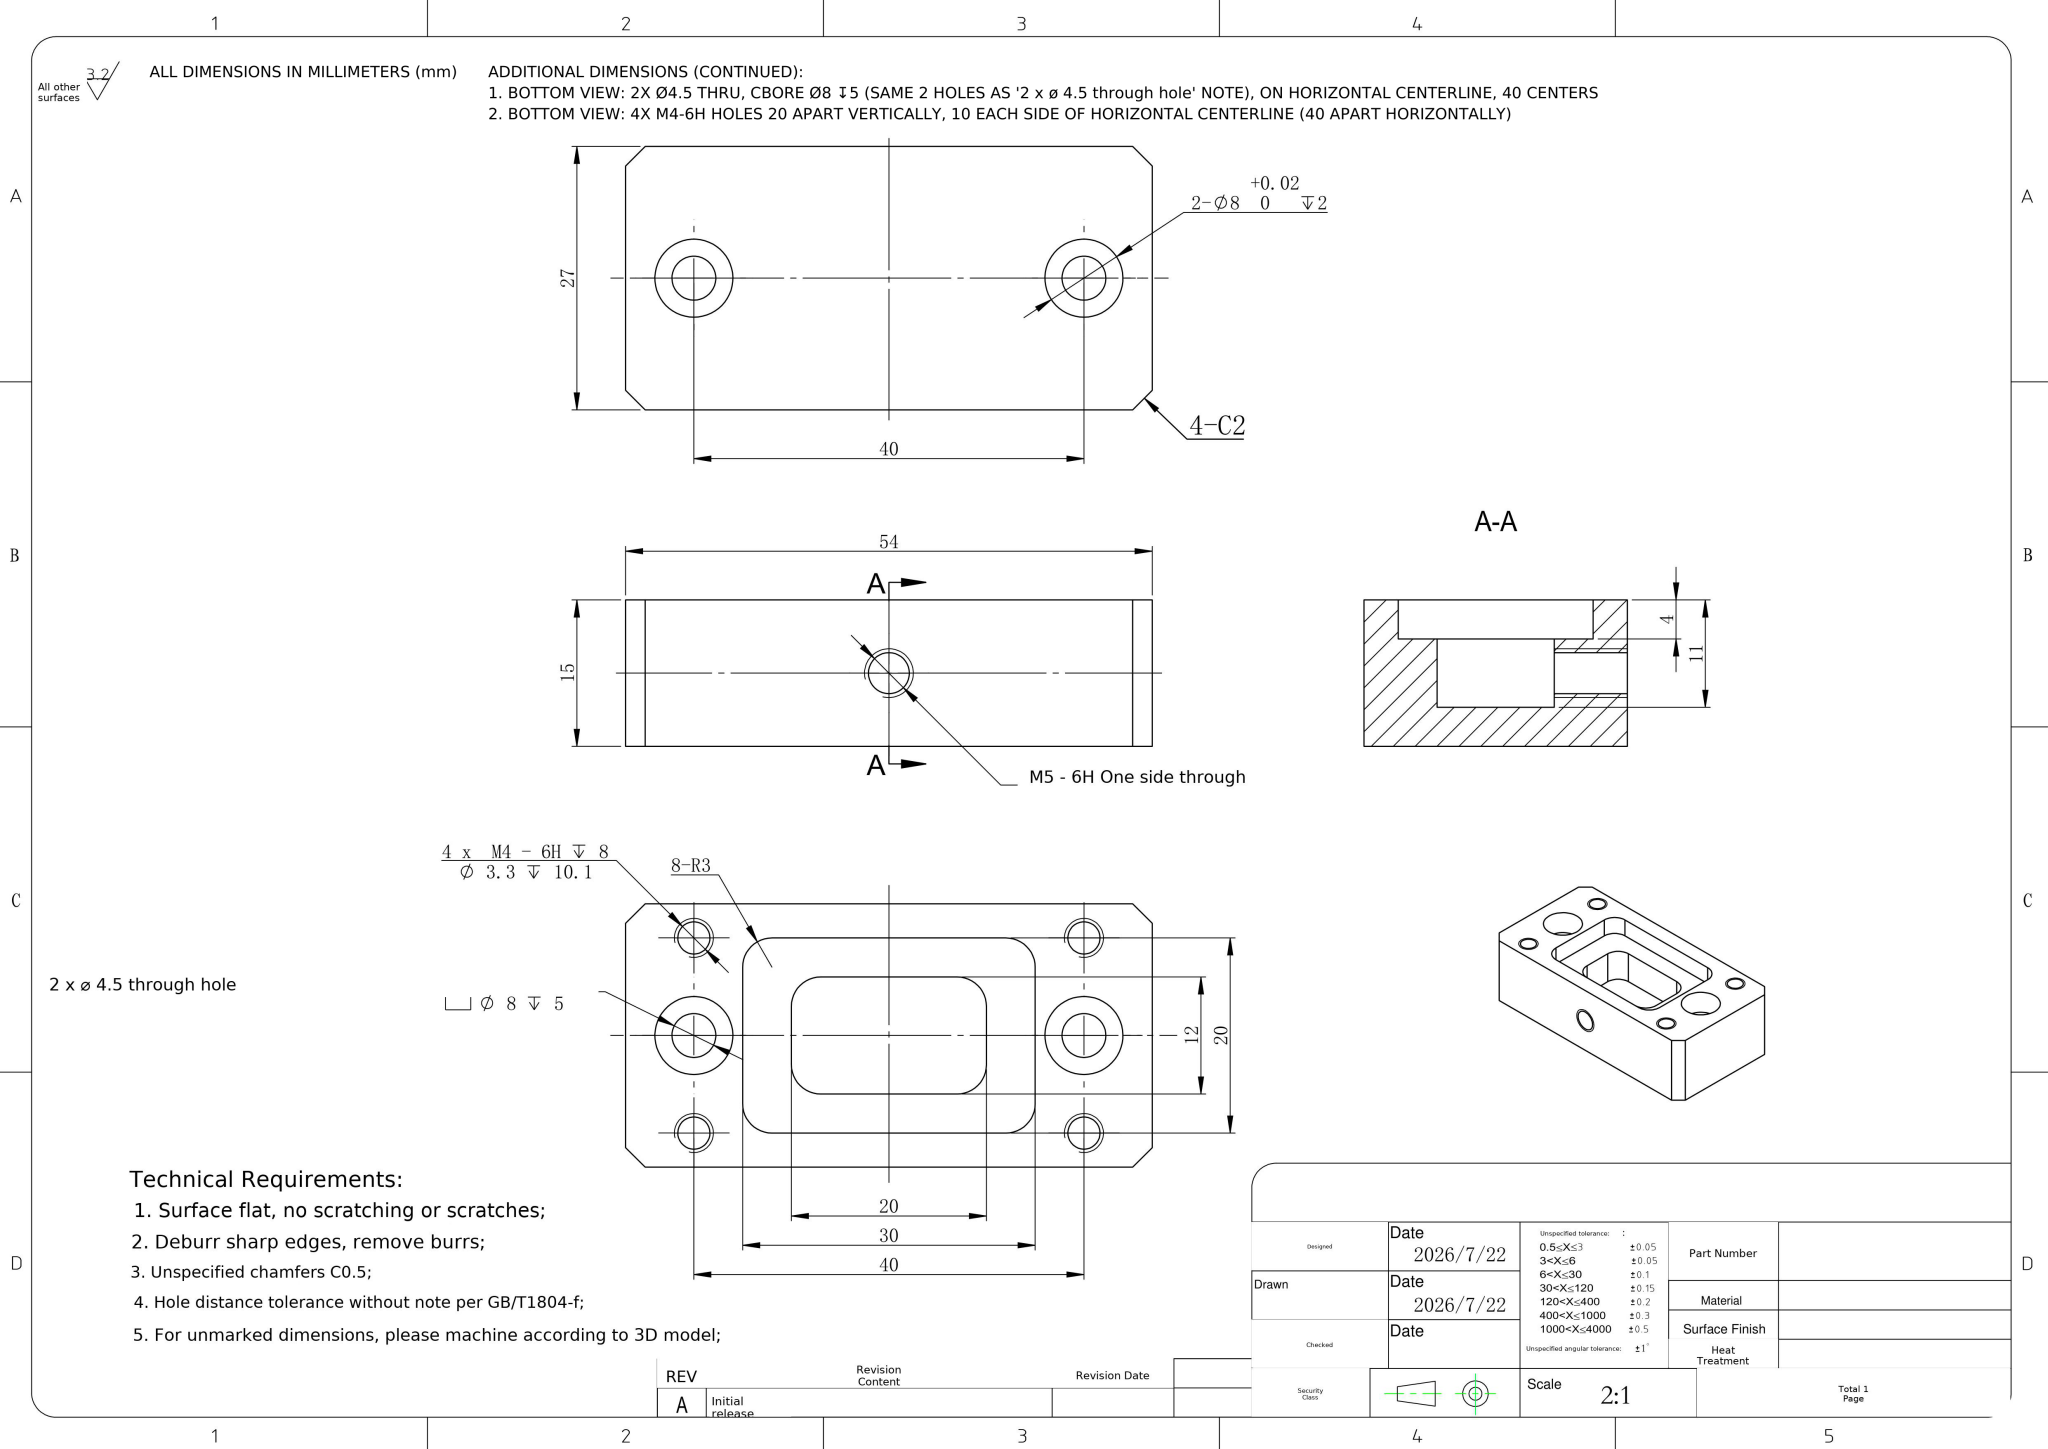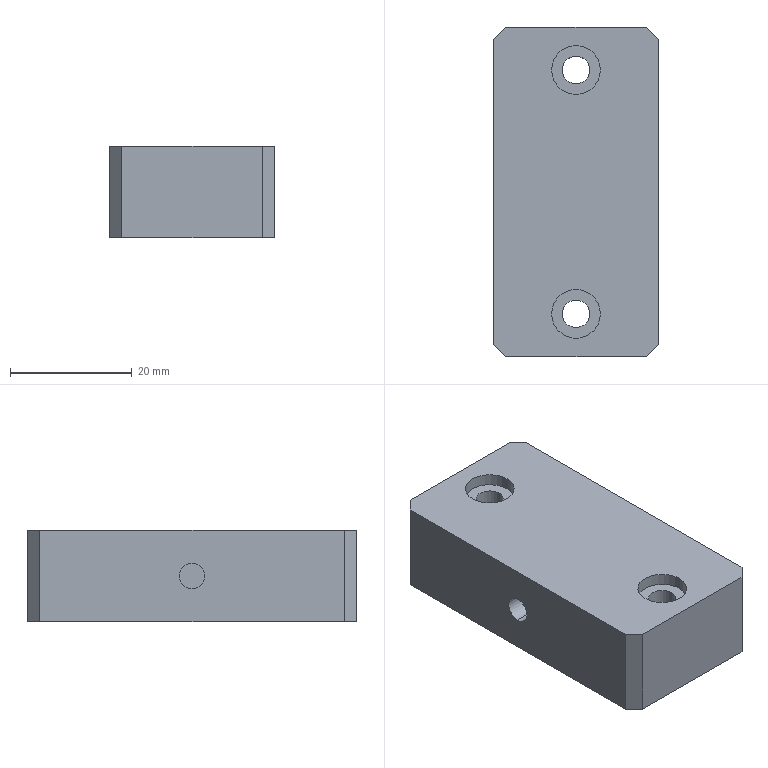Part | NX | mm | 1 solid | 62 faces | box 27 x 54 x 15 mm | volume 16336 mm3 | cylinder 30 | plane 24 | cone 8 | commonest cylinder face diameters 8 x8 3.3 x8 6 x8 4.5 x4 4.2 x2